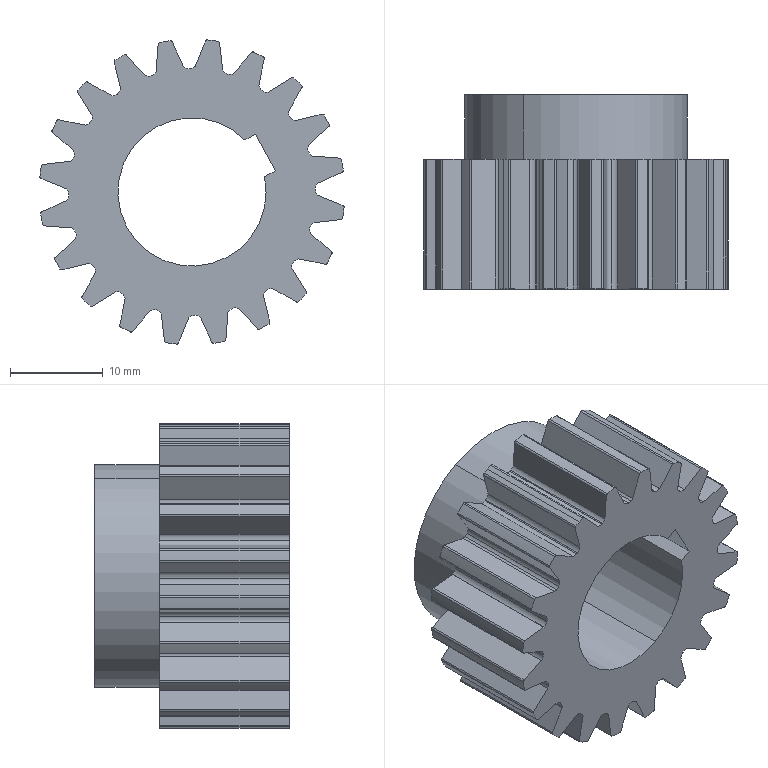Component | SolidWorks | Pignon 20T-1 | 1 solid | 236 faces | box 32.84 x 21 x 32.84 mm | volume 8745 mm3 | cylinder 152 | plane 44 | spline 40 | commonest cylinder face diameters 1.771 x86 0.4 x40 33 x21 16 x3 24 x2